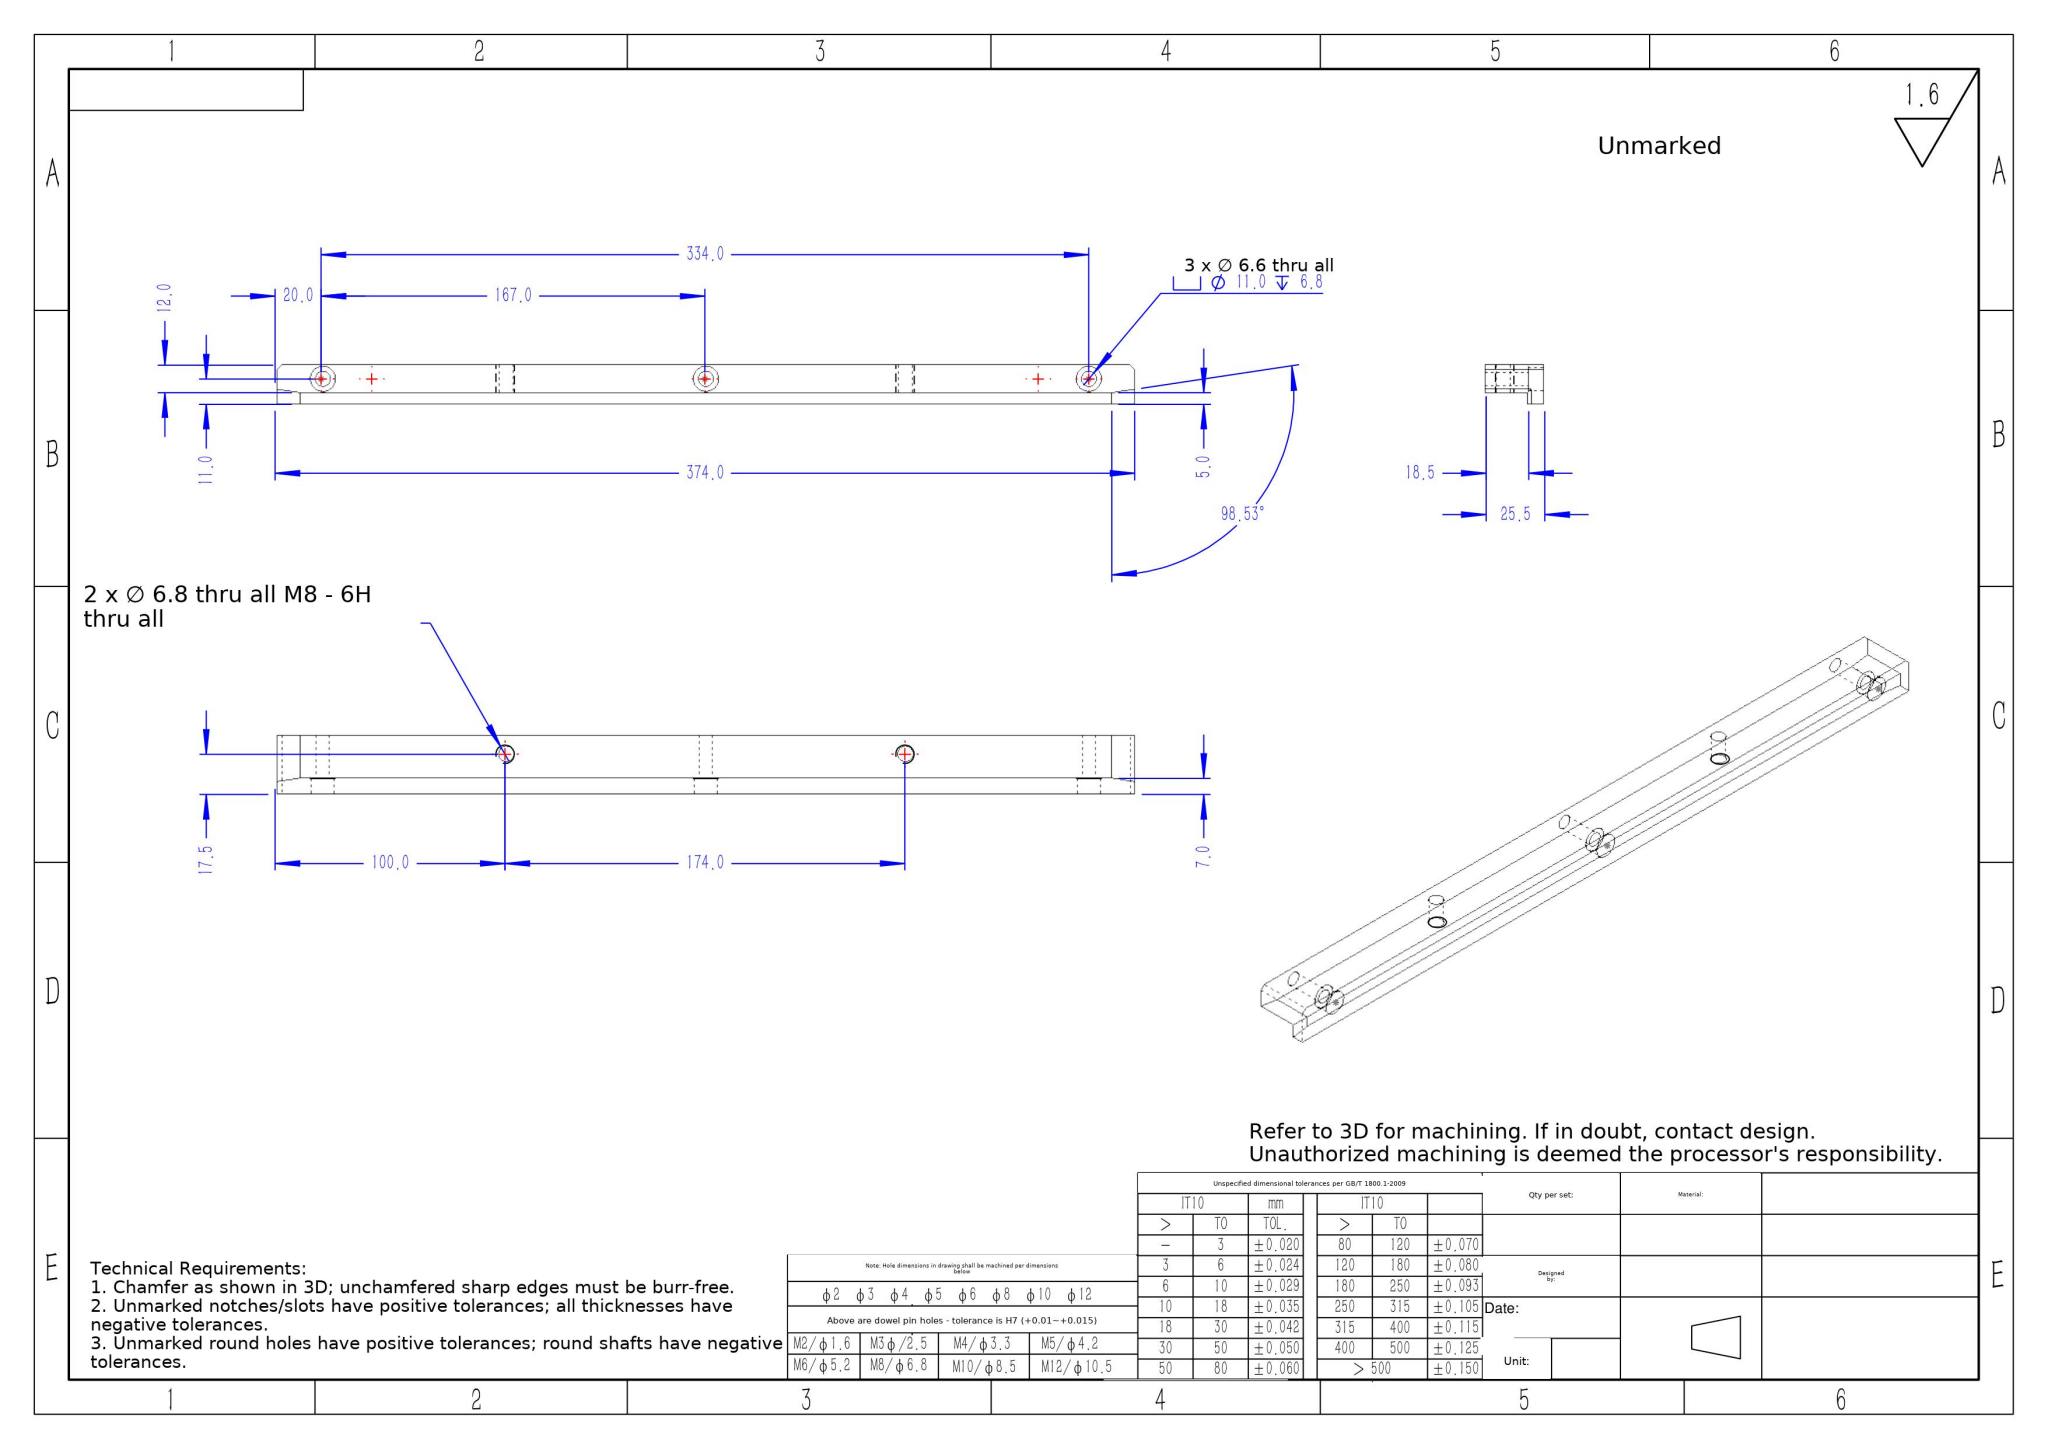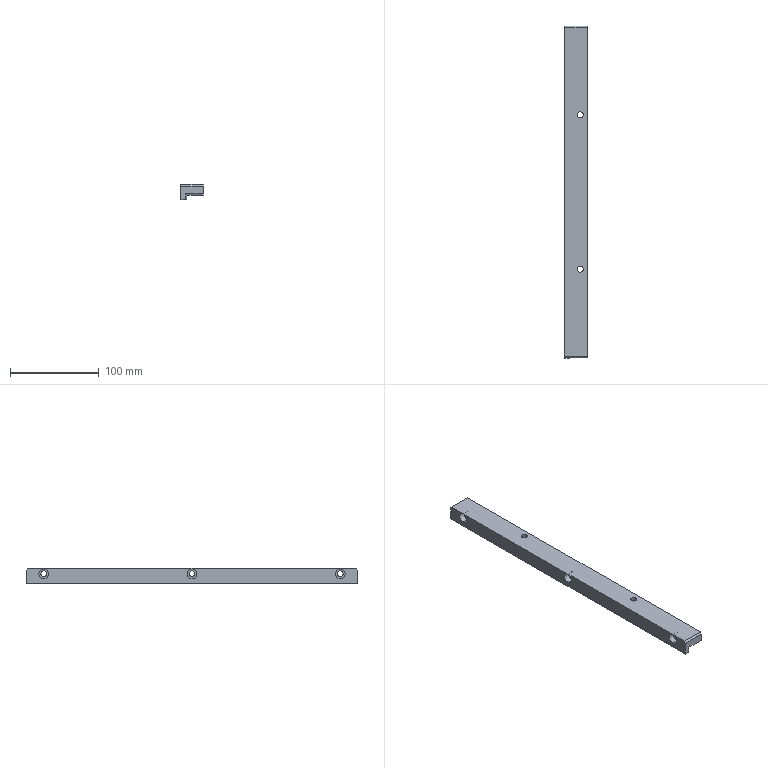Part | SolidWorks | mm | 1 solid | 33 faces | box 25.5 x 374 x 17 mm | volume 122335 mm3 | plane 17 | cylinder 16 | commonest cylinder face diameters 11 x6 6.6 x6 6.8 x4
STEP:
#1=CARTESIAN_POINT('',(14.,83.6,17.));
#2=VERTEX_POINT('',#1);
#3=CARTESIAN_POINT('',(14.,90.4,17.));
#4=VERTEX_POINT('',#3);
#5=CARTESIAN_POINT('',(14.,87.,17.));
#6=DIRECTION('',(0.,-0.,-1.));
#7=DIRECTION('',(0.,1.,0.));
#8=AXIS2_PLACEMENT_3D('',#5,#6,#7);
#9=CIRCLE('',#8,3.4);
#10=EDGE_CURVE('',#2,#4,#9,.T.);
#11=ORIENTED_EDGE('',*,*,#10,.F.);
#12=CARTESIAN_POINT('',(14.,83.6,5.));
#13=VERTEX_POINT('',#12);
#14=CARTESIAN_POINT('',(14.,83.6,5.));
#15=DIRECTION('',(0.,-0.,-1.));
#16=VECTOR('',#15,1000.);
#17=LINE('',#14,#16);
#18=EDGE_CURVE('',#2,#13,#17,.T.);
#19=ORIENTED_EDGE('',*,*,#18,.T.);
#20=CARTESIAN_POINT('',(14.,90.4,5.));
#21=VERTEX_POINT('',#20);
#22=CARTESIAN_POINT('',(14.,87.,5.));
#23=DIRECTION('',(0.,-0.,-1.));
#24=DIRECTION('',(0.,1.,0.));
#25=AXIS2_PLACEMENT_3D('',#22,#23,#24);
#26=CIRCLE('',#25,3.4);
#27=EDGE_CURVE('',#13,#21,#26,.T.);
#28=ORIENTED_EDGE('',*,*,#27,.T.);
#29=CARTESIAN_POINT('',(14.,90.4,5.));
#30=DIRECTION('',(0.,-0.,-1.));
#31=VECTOR('',#30,1000.);
#32=LINE('',#29,#31);
#33=EDGE_CURVE('',#4,#21,#32,.T.);
#34=ORIENTED_EDGE('',*,*,#33,.F.);
#35=EDGE_LOOP('',(#11,#19,#28,#34));
#36=FACE_OUTER_BOUND('',#35,.T.);
#37=CARTESIAN_POINT('',(14.,87.,5.));
#38=DIRECTION('',(0.,-0.,-1.));
#39=DIRECTION('',(0.,1.,0.));
#40=AXIS2_PLACEMENT_3D('',#37,#38,#39);
#41=CYLINDRICAL_SURFACE('',#40,3.4);
#42=ADVANCED_FACE('',(#36),#41,.F.);
#43=CARTESIAN_POINT('',(14.,-90.4,17.));
#44=VERTEX_POINT('',#43);
#45=CARTESIAN_POINT('',(14.,-83.6,17.));
#46=VERTEX_POINT('',#45);
#47=CARTESIAN_POINT('',(14.,-87.,17.));
#48=DIRECTION('',(0.,0.,-1.));
#49=DIRECTION('',(0.,1.,0.));
#50=AXIS2_PLACEMENT_3D('',#47,#48,#49);
#51=CIRCLE('',#50,3.4);
#52=EDGE_CURVE('',#44,#46,#51,.T.);
#53=ORIENTED_EDGE('',*,*,#52,.F.);
#54=CARTESIAN_POINT('',(14.,-90.4,5.));
#55=VERTEX_POINT('',#54);
#56=CARTESIAN_POINT('',(14.,-90.4,5.));
#57=DIRECTION('',(0.,0.,-1.));
#58=VECTOR('',#57,1000.);
#59=LINE('',#56,#58);
#60=EDGE_CURVE('',#44,#55,#59,.T.);
#61=ORIENTED_EDGE('',*,*,#60,.T.);
#62=CARTESIAN_POINT('',(14.,-83.6,5.));
#63=VERTEX_POINT('',#62);
#64=CARTESIAN_POINT('',(14.,-87.,5.));
#65=DIRECTION('',(0.,0.,-1.));
#66=DIRECTION('',(0.,1.,0.));
#67=AXIS2_PLACEMENT_3D('',#64,#65,#66);
#68=CIRCLE('',#67,3.4);
#69=EDGE_CURVE('',#55,#63,#68,.T.);
#70=ORIENTED_EDGE('',*,*,#69,.T.);
#71=CARTESIAN_POINT('',(14.,-83.6,5.));
#72=DIRECTION('',(0.,0.,-1.));
#73=VECTOR('',#72,1000.);
#74=LINE('',#71,#73);
#75=EDGE_CURVE('',#46,#63,#74,.T.);
#76=ORIENTED_EDGE('',*,*,#75,.F.);
#77=EDGE_LOOP('',(#53,#61,#70,#76));
#78=FACE_OUTER_BOUND('',#77,.T.);
#79=CARTESIAN_POINT('',(14.,-87.,5.));
#80=DIRECTION('',(0.,0.,-1.));
#81=DIRECTION('',(0.,1.,0.));
#82=AXIS2_PLACEMENT_3D('',#79,#80,#81);
#83=CYLINDRICAL_SURFACE('',#82,3.4);
#84=ADVANCED_FACE('',(#78),#83,.F.);
#85=CARTESIAN_POINT('',(3.3,-167.,5.5));
#86=VERTEX_POINT('',#85);
#87=CARTESIAN_POINT('',(3.3,-167.,16.5));
#88=VERTEX_POINT('',#87);
#89=CARTESIAN_POINT('',(3.3,-167.,11.));
#90=DIRECTION('',(-1.,0.,0.));
#91=DIRECTION('',(0.,0.,1.));
#92=AXIS2_PLACEMENT_3D('',#89,#90,#91);
#93=CIRCLE('',#92,5.5);
#94=EDGE_CURVE('',#86,#88,#93,.T.);
#95=ORIENTED_EDGE('',*,*,#94,.F.);
#96=CARTESIAN_POINT('',(-3.5,-167.,5.5));
#97=VERTEX_POINT('',#96);
#98=CARTESIAN_POINT('',(-3.5,-167.,5.5));
#99=DIRECTION('',(-1.,0.,0.));
#100=VECTOR('',#99,1000.);
#101=LINE('',#98,#100);
#102=EDGE_CURVE('',#86,#97,#101,.T.);
#103=ORIENTED_EDGE('',*,*,#102,.T.);
#104=CARTESIAN_POINT('',(-3.5,-167.,16.5));
#105=VERTEX_POINT('',#104);
#106=CARTESIAN_POINT('',(-3.5,-167.,11.));
#107=DIRECTION('',(-1.,0.,0.));
#108=DIRECTION('',(0.,0.,1.));
#109=AXIS2_PLACEMENT_3D('',#106,#107,#108);
#110=CIRCLE('',#109,5.5);
#111=EDGE_CURVE('',#97,#105,#110,.T.);
#112=ORIENTED_EDGE('',*,*,#111,.T.);
#113=CARTESIAN_POINT('',(-3.5,-167.,16.5));
#114=DIRECTION('',(-1.,0.,0.));
#115=VECTOR('',#114,1000.);
#116=LINE('',#113,#115);
#117=EDGE_CURVE('',#88,#105,#116,.T.);
#118=ORIENTED_EDGE('',*,*,#117,.F.);
#119=EDGE_LOOP('',(#95,#103,#112,#118));
#120=FACE_OUTER_BOUND('',#119,.T.);
#121=CARTESIAN_POINT('',(-3.5,-167.,11.));
#122=DIRECTION('',(-1.,0.,0.));
#123=DIRECTION('',(0.,0.,1.));
#124=AXIS2_PLACEMENT_3D('',#121,#122,#123);
#125=CYLINDRICAL_SURFACE('',#124,5.5);
#126=ADVANCED_FACE('',(#120),#125,.F.);
#127=CARTESIAN_POINT('',(22.,-167.,7.7));
#128=VERTEX_POINT('',#127);
#129=CARTESIAN_POINT('',(22.,-167.,14.3));
#130=VERTEX_POINT('',#129);
#131=CARTESIAN_POINT('',(22.,-167.,11.));
#132=DIRECTION('',(-1.,0.,0.));
#133=DIRECTION('',(0.,0.,1.));
#134=AXIS2_PLACEMENT_3D('',#131,#132,#133);
#135=CIRCLE('',#134,3.3);
#136=EDGE_CURVE('',#128,#130,#135,.T.);
#137=ORIENTED_EDGE('',*,*,#136,.F.);
#138=CARTESIAN_POINT('',(3.3,-167.,7.7));
#139=VERTEX_POINT('',#138);
#140=CARTESIAN_POINT('',(-3.5,-167.,7.7));
#141=DIRECTION('',(-1.,0.,0.));
#142=VECTOR('',#141,1000.);
#143=LINE('',#140,#142);
#144=EDGE_CURVE('',#128,#139,#143,.T.);
#145=ORIENTED_EDGE('',*,*,#144,.T.);
#146=CARTESIAN_POINT('',(3.3,-167.,14.3));
#147=VERTEX_POINT('',#146);
#148=CARTESIAN_POINT('',(3.3,-167.,11.));
#149=DIRECTION('',(-1.,0.,0.));
#150=DIRECTION('',(0.,0.,1.));
#151=AXIS2_PLACEMENT_3D('',#148,#149,#150);
#152=CIRCLE('',#151,3.3);
#153=EDGE_CURVE('',#139,#147,#152,.T.);
#154=ORIENTED_EDGE('',*,*,#153,.T.);
#155=CARTESIAN_POINT('',(-3.5,-167.,14.3));
#156=DIRECTION('',(-1.,0.,0.));
#157=VECTOR('',#156,1000.);
#158=LINE('',#155,#157);
#159=EDGE_CURVE('',#130,#147,#158,.T.);
#160=ORIENTED_EDGE('',*,*,#159,.F.);
#161=EDGE_LOOP('',(#137,#145,#154,#160));
#162=FACE_OUTER_BOUND('',#161,.T.);
#163=CARTESIAN_POINT('',(-3.5,-167.,11.));
#164=DIRECTION('',(-1.,0.,0.));
#165=DIRECTION('',(0.,0.,1.));
#166=AXIS2_PLACEMENT_3D('',#163,#164,#165);
#167=CYLINDRICAL_SURFACE('',#166,3.3);
#168=ADVANCED_FACE('',(#162),#167,.F.);
#169=CARTESIAN_POINT('',(3.3,0.,5.5));
#170=VERTEX_POINT('',#169);
#171=CARTESIAN_POINT('',(3.3,0.,16.5));
#172=VERTEX_POINT('',#171);
#173=CARTESIAN_POINT('',(3.3,0.,11.));
#174=DIRECTION('',(-1.,0.,0.));
#175=DIRECTION('',(0.,0.,1.));
#176=AXIS2_PLACEMENT_3D('',#173,#174,#175);
#177=CIRCLE('',#176,5.5);
#178=EDGE_CURVE('',#170,#172,#177,.T.);
#179=ORIENTED_EDGE('',*,*,#178,.F.);
#180=CARTESIAN_POINT('',(-3.5,0.,5.5));
#181=VERTEX_POINT('',#180);
#182=CARTESIAN_POINT('',(-3.5,0.,5.5));
#183=DIRECTION('',(-1.,0.,0.));
#184=VECTOR('',#183,1000.);
#185=LINE('',#182,#184);
#186=EDGE_CURVE('',#170,#181,#185,.T.);
#187=ORIENTED_EDGE('',*,*,#186,.T.);
#188=CARTESIAN_POINT('',(-3.5,0.,16.5));
#189=VERTEX_POINT('',#188);
#190=CARTESIAN_POINT('',(-3.5,0.,11.));
#191=DIRECTION('',(-1.,0.,0.));
#192=DIRECTION('',(0.,0.,1.));
#193=AXIS2_PLACEMENT_3D('',#190,#191,#192);
#194=CIRCLE('',#193,5.5);
#195=EDGE_CURVE('',#181,#189,#194,.T.);
#196=ORIENTED_EDGE('',*,*,#195,.T.);
#197=CARTESIAN_POINT('',(-3.5,0.,16.5));
#198=DIRECTION('',(-1.,0.,0.));
#199=VECTOR('',#198,1000.);
#200=LINE('',#197,#199);
#201=EDGE_CURVE('',#172,#189,#200,.T.);
#202=ORIENTED_EDGE('',*,*,#201,.F.);
#203=EDGE_LOOP('',(#179,#187,#196,#202));
#204=FACE_OUTER_BOUND('',#203,.T.);
#205=CARTESIAN_POINT('',(-3.5,0.,11.));
#206=DIRECTION('',(-1.,0.,0.));
#207=DIRECTION('',(0.,0.,1.));
#208=AXIS2_PLACEMENT_3D('',#205,#206,#207);
#209=CYLINDRICAL_SURFACE('',#208,5.5);
#210=ADVANCED_FACE('',(#204),#209,.F.);
#211=CARTESIAN_POINT('',(22.,0.,7.7));
#212=VERTEX_POINT('',#211);
#213=CARTESIAN_POINT('',(22.,0.,14.3));
#214=VERTEX_POINT('',#213);
#215=CARTESIAN_POINT('',(22.,0.,11.));
#216=DIRECTION('',(-1.,0.,0.));
#217=DIRECTION('',(0.,0.,1.));
#218=AXIS2_PLACEMENT_3D('',#215,#216,#217);
#219=CIRCLE('',#218,3.3);
#220=EDGE_CURVE('',#212,#214,#219,.T.);
#221=ORIENTED_EDGE('',*,*,#220,.F.);
#222=CARTESIAN_POINT('',(3.3,0.,7.7));
#223=VERTEX_POINT('',#222);
#224=CARTESIAN_POINT('',(-3.5,0.,7.7));
#225=DIRECTION('',(-1.,0.,0.));
#226=VECTOR('',#225,1000.);
#227=LINE('',#224,#226);
#228=EDGE_CURVE('',#212,#223,#227,.T.);
#229=ORIENTED_EDGE('',*,*,#228,.T.);
#230=CARTESIAN_POINT('',(3.3,0.,14.3));
#231=VERTEX_POINT('',#230);
#232=CARTESIAN_POINT('',(3.3,0.,11.));
#233=DIRECTION('',(-1.,0.,0.));
#234=DIRECTION('',(0.,0.,1.));
#235=AXIS2_PLACEMENT_3D('',#232,#233,#234);
#236=CIRCLE('',#235,3.3);
#237=EDGE_CURVE('',#223,#231,#236,.T.);
#238=ORIENTED_EDGE('',*,*,#237,.T.);
#239=CARTESIAN_POINT('',(-3.5,0.,14.3));
#240=DIRECTION('',(-1.,0.,0.));
#241=VECTOR('',#240,1000.);
#242=LINE('',#239,#241);
#243=EDGE_CURVE('',#214,#231,#242,.T.);
#244=ORIENTED_EDGE('',*,*,#243,.F.);
#245=EDGE_LOOP('',(#221,#229,#238,#244));
#246=FACE_OUTER_BOUND('',#245,.T.);
#247=CARTESIAN_POINT('',(-3.5,0.,11.));
#248=DIRECTION('',(-1.,0.,0.));
#249=DIRECTION('',(0.,0.,1.));
#250=AXIS2_PLACEMENT_3D('',#247,#248,#249);
#251=CYLINDRICAL_SURFACE('',#250,3.3);
#252=ADVANCED_FACE('',(#246),#251,.F.);
#253=CARTESIAN_POINT('',(3.3,167.,5.5));
#254=VERTEX_POINT('',#253);
#255=CARTESIAN_POINT('',(3.3,167.,16.5));
#256=VERTEX_POINT('',#255);
#257=CARTESIAN_POINT('',(3.3,167.,11.));
#258=DIRECTION('',(-1.,0.,0.));
#259=DIRECTION('',(0.,0.,1.));
#260=AXIS2_PLACEMENT_3D('',#257,#258,#259);
#261=CIRCLE('',#260,5.5);
#262=EDGE_CURVE('',#254,#256,#261,.T.);
#263=ORIENTED_EDGE('',*,*,#262,.F.);
#264=CARTESIAN_POINT('',(-3.5,167.,5.5));
#265=VERTEX_POINT('',#264);
#266=CARTESIAN_POINT('',(-3.5,167.,5.5));
#267=DIRECTION('',(-1.,0.,0.));
#268=VECTOR('',#267,1000.);
#269=LINE('',#266,#268);
#270=EDGE_CURVE('',#254,#265,#269,.T.);
#271=ORIENTED_EDGE('',*,*,#270,.T.);
#272=CARTESIAN_POINT('',(-3.5,167.,16.5));
#273=VERTEX_POINT('',#272);
#274=CARTESIAN_POINT('',(-3.5,167.,11.));
#275=DIRECTION('',(-1.,0.,0.));
#276=DIRECTION('',(0.,0.,1.));
#277=AXIS2_PLACEMENT_3D('',#274,#275,#276);
#278=CIRCLE('',#277,5.5);
#279=EDGE_CURVE('',#265,#273,#278,.T.);
#280=ORIENTED_EDGE('',*,*,#279,.T.);
#281=CARTESIAN_POINT('',(-3.5,167.,16.5));
#282=DIRECTION('',(-1.,0.,0.));
#283=VECTOR('',#282,1000.);
#284=LINE('',#281,#283);
#285=EDGE_CURVE('',#256,#273,#284,.T.);
#286=ORIENTED_EDGE('',*,*,#285,.F.);
#287=EDGE_LOOP('',(#263,#271,#280,#286));
#288=FACE_OUTER_BOUND('',#287,.T.);
#289=CARTESIAN_POINT('',(-3.5,167.,11.));
#290=DIRECTION('',(-1.,0.,0.));
#291=DIRECTION('',(0.,0.,1.));
#292=AXIS2_PLACEMENT_3D('',#289,#290,#291);
#293=CYLINDRICAL_SURFACE('',#292,5.5);
#294=ADVANCED_FACE('',(#288),#293,.F.);
#295=CARTESIAN_POINT('',(22.,167.,7.7));
#296=VERTEX_POINT('',#295);
#297=CARTESIAN_POINT('',(22.,167.,14.3));
#298=VERTEX_POINT('',#297);
#299=CARTESIAN_POINT('',(22.,167.,11.));
#300=DIRECTION('',(-1.,0.,0.));
#301=DIRECTION('',(0.,0.,1.));
#302=AXIS2_PLACEMENT_3D('',#299,#300,#301);
#303=CIRCLE('',#302,3.3);
#304=EDGE_CURVE('',#296,#298,#303,.T.);
#305=ORIENTED_EDGE('',*,*,#304,.F.);
#306=CARTESIAN_POINT('',(3.3,167.,7.7));
#307=VERTEX_POINT('',#306);
#308=CARTESIAN_POINT('',(-3.5,167.,7.7));
#309=DIRECTION('',(-1.,0.,0.));
#310=VECTOR('',#309,1000.);
#311=LINE('',#308,#310);
#312=EDGE_CURVE('',#296,#307,#311,.T.);
#313=ORIENTED_EDGE('',*,*,#312,.T.);
#314=CARTESIAN_POINT('',(3.3,167.,14.3));
#315=VERTEX_POINT('',#314);
#316=CARTESIAN_POINT('',(3.3,167.,11.));
#317=DIRECTION('',(-1.,0.,0.));
#318=DIRECTION('',(0.,0.,1.));
#319=AXIS2_PLACEMENT_3D('',#316,#317,#318);
#320=CIRCLE('',#319,3.3);
#321=EDGE_CURVE('',#307,#315,#320,.T.);
#322=ORIENTED_EDGE('',*,*,#321,.T.);
#323=CARTESIAN_POINT('',(-3.5,167.,14.3));
#324=DIRECTION('',(-1.,0.,0.));
#325=VECTOR('',#324,1000.);
#326=LINE('',#323,#325);
#327=EDGE_CURVE('',#298,#315,#326,.T.);
#328=ORIENTED_EDGE('',*,*,#327,.F.);
#329=EDGE_LOOP('',(#305,#313,#322,#328));
#330=FACE_OUTER_BOUND('',#329,.T.);
#331=CARTESIAN_POINT('',(-3.5,167.,11.));
#332=DIRECTION('',(-1.,0.,0.));
#333=DIRECTION('',(0.,0.,1.));
#334=AXIS2_PLACEMENT_3D('',#331,#332,#333);
#335=CYLINDRICAL_SURFACE('',#334,3.3);
#336=ADVANCED_FACE('',(#330),#335,.F.);
#337=CARTESIAN_POINT('',(3.5,-177.,0.));
#338=VERTEX_POINT('',#337);
#339=CARTESIAN_POINT('',(3.5,177.,0.));
#340=VERTEX_POINT('',#339);
#341=CARTESIAN_POINT('',(3.5,-187.,0.));
#342=DIRECTION('',(0.,1.,0.));
#343=VECTOR('',#342,1000.);
#344=LINE('',#341,#343);
#345=EDGE_CURVE('',#338,#340,#344,.T.);
#346=ORIENTED_EDGE('',*,*,#345,.T.);
#347=CARTESIAN_POINT('',(3.5,177.,5.));
#348=VERTEX_POINT('',#347);
#349=CARTESIAN_POINT('',(3.5,177.,17.));
#350=DIRECTION('',(0.,0.,1.));
#351=VECTOR('',#350,1000.);
#352=LINE('',#349,#351);
#353=EDGE_CURVE('',#340,#348,#352,.T.);
#354=ORIENTED_EDGE('',*,*,#353,.T.);
#355=CARTESIAN_POINT('',(3.5,-177.,5.));
#356=VERTEX_POINT('',#355);
#357=CARTESIAN_POINT('',(3.5,187.,5.));
#358=DIRECTION('',(0.,1.,0.));
#359=VECTOR('',#358,1000.);
#360=LINE('',#357,#359);
#361=EDGE_CURVE('',#356,#348,#360,.T.);
#362=ORIENTED_EDGE('',*,*,#361,.F.);
#363=CARTESIAN_POINT('',(3.5,-177.,17.));
#364=DIRECTION('',(0.,0.,-1.));
#365=VECTOR('',#364,1000.);
#366=LINE('',#363,#365);
#367=EDGE_CURVE('',#356,#338,#366,.T.);
#368=ORIENTED_EDGE('',*,*,#367,.T.);
#369=EDGE_LOOP('',(#346,#354,#362,#368));
#370=FACE_OUTER_BOUND('',#369,.T.);
#371=CARTESIAN_POINT('',(3.5,-187.,17.));
#372=DIRECTION('',(-1.,0.,0.));
#373=DIRECTION('',(0.,0.,1.));
#374=AXIS2_PLACEMENT_3D('',#371,#372,#373);
#375=PLANE('',#374);
#376=ADVANCED_FACE('',(#370),#375,.F.);
#377=CARTESIAN_POINT('',(-3.5,187.,15.));
#378=VERTEX_POINT('',#377);
#379=CARTESIAN_POINT('',(-3.5,187.,0.));
#380=VERTEX_POINT('',#379);
#381=CARTESIAN_POINT('',(-3.5,187.,17.));
#382=DIRECTION('',(0.,0.,-1.));
#383=VECTOR('',#382,1000.);
#384=LINE('',#381,#383);
#385=EDGE_CURVE('',#378,#380,#384,.T.);
#386=ORIENTED_EDGE('',*,*,#385,.F.);
#387=CARTESIAN_POINT('',(22.,187.,15.));
#388=VERTEX_POINT('',#387);
#389=CARTESIAN_POINT('',(-3.5,187.,15.));
#390=DIRECTION('',(1.,0.,0.));
#391=VECTOR('',#390,1000.);
#392=LINE('',#389,#391);
#393=EDGE_CURVE('',#378,#388,#392,.T.);
#394=ORIENTED_EDGE('',*,*,#393,.T.);
#395=CARTESIAN_POINT('',(22.,187.,6.5));
#396=VERTEX_POINT('',#395);
#397=CARTESIAN_POINT('',(22.,187.,17.));
#398=DIRECTION('',(0.,0.,1.));
#399=VECTOR('',#398,1000.);
#400=LINE('',#397,#399);
#401=EDGE_CURVE('',#396,#388,#400,.T.);
#402=ORIENTED_EDGE('',*,*,#401,.F.);
#403=CARTESIAN_POINT('',(2.,187.,6.5));
#404=VERTEX_POINT('',#403);
#405=CARTESIAN_POINT('',(-3.5,187.,6.5));
#406=DIRECTION('',(-1.,0.,0.));
#407=VECTOR('',#406,1000.);
#408=LINE('',#405,#407);
#409=EDGE_CURVE('',#396,#404,#408,.T.);
#410=ORIENTED_EDGE('',*,*,#409,.T.);
#411=CARTESIAN_POINT('',(2.,187.,0.));
#412=VERTEX_POINT('',#411);
#413=CARTESIAN_POINT('',(2.,187.,17.));
#414=DIRECTION('',(0.,0.,-1.));
#415=VECTOR('',#414,1000.);
#416=LINE('',#413,#415);
#417=EDGE_CURVE('',#404,#412,#416,.T.);
#418=ORIENTED_EDGE('',*,*,#417,.T.);
#419=CARTESIAN_POINT('',(-3.5,187.,0.));
#420=DIRECTION('',(-1.,0.,0.));
#421=VECTOR('',#420,1000.);
#422=LINE('',#419,#421);
#423=EDGE_CURVE('',#412,#380,#422,.T.);
#424=ORIENTED_EDGE('',*,*,#423,.T.);
#425=EDGE_LOOP('',(#386,#394,#402,#410,#418,#424));
#426=FACE_OUTER_BOUND('',#425,.T.);
#427=CARTESIAN_POINT('',(-3.5,187.,17.));
#428=DIRECTION('',(0.,-1.,0.));
#429=DIRECTION('',(0.,0.,-1.));
#430=AXIS2_PLACEMENT_3D('',#427,#428,#429);
#431=PLANE('',#430);
#432=ADVANCED_FACE('',(#426),#431,.F.);
#433=CARTESIAN_POINT('',(-3.5,-167.,11.));
#434=DIRECTION('',(-1.,0.,0.));
#435=DIRECTION('',(0.,0.,1.));
#436=AXIS2_PLACEMENT_3D('',#433,#434,#435);
#437=CIRCLE('',#436,5.5);
#438=EDGE_CURVE('',#105,#97,#437,.T.);
#439=ORIENTED_EDGE('',*,*,#438,.F.);
#440=ORIENTED_EDGE('',*,*,#111,.F.);
#441=EDGE_LOOP('',(#439,#440));
#442=FACE_BOUND('',#441,.T.);
#443=CARTESIAN_POINT('',(-3.5,0.,11.));
#444=DIRECTION('',(-1.,0.,0.));
#445=DIRECTION('',(0.,0.,1.));
#446=AXIS2_PLACEMENT_3D('',#443,#444,#445);
#447=CIRCLE('',#446,5.5);
#448=EDGE_CURVE('',#189,#181,#447,.T.);
#449=ORIENTED_EDGE('',*,*,#448,.F.);
#450=ORIENTED_EDGE('',*,*,#195,.F.);
#451=EDGE_LOOP('',(#449,#450));
#452=FACE_BOUND('',#451,.T.);
#453=CARTESIAN_POINT('',(-3.5,167.,11.));
#454=DIRECTION('',(-1.,0.,0.));
#455=DIRECTION('',(0.,0.,1.));
#456=AXIS2_PLACEMENT_3D('',#453,#454,#455);
#457=CIRCLE('',#456,5.5);
#458=EDGE_CURVE('',#273,#265,#457,.T.);
#459=ORIENTED_EDGE('',*,*,#458,.F.);
#460=ORIENTED_EDGE('',*,*,#279,.F.);
#461=EDGE_LOOP('',(#459,#460));
#462=FACE_BOUND('',#461,.T.);
#463=CARTESIAN_POINT('',(-3.5,-187.,15.));
#464=VERTEX_POINT('',#463);
#465=CARTESIAN_POINT('',(-3.5,-187.,0.));
#466=VERTEX_POINT('',#465);
#467=CARTESIAN_POINT('',(-3.5,-187.,17.));
#468=DIRECTION('',(0.,0.,-1.));
#469=VECTOR('',#468,1000.);
#470=LINE('',#467,#469);
#471=EDGE_CURVE('',#464,#466,#470,.T.);
#472=ORIENTED_EDGE('',*,*,#471,.F.);
#473=CARTESIAN_POINT('',(-3.5,-185.,17.));
#474=VERTEX_POINT('',#473);
#475=CARTESIAN_POINT('',(-3.5,-185.,17.));
#476=DIRECTION('',(0.,0.7071,0.7071));
#477=VECTOR('',#476,1000.);
#478=LINE('',#475,#477);
#479=EDGE_CURVE('',#464,#474,#478,.T.);
#480=ORIENTED_EDGE('',*,*,#479,.T.);
#481=CARTESIAN_POINT('',(-3.5,185.,17.));
#482=VERTEX_POINT('',#481);
#483=CARTESIAN_POINT('',(-3.5,-187.,17.));
#484=DIRECTION('',(0.,-1.,0.));
#485=VECTOR('',#484,1000.);
#486=LINE('',#483,#485);
#487=EDGE_CURVE('',#482,#474,#486,.T.);
#488=ORIENTED_EDGE('',*,*,#487,.F.);
#489=CARTESIAN_POINT('',(-3.5,185.,17.));
#490=DIRECTION('',(0.,0.7071,-0.7071));
#491=VECTOR('',#490,1000.);
#492=LINE('',#489,#491);
#493=EDGE_CURVE('',#482,#378,#492,.T.);
#494=ORIENTED_EDGE('',*,*,#493,.T.);
#495=ORIENTED_EDGE('',*,*,#385,.T.);
#496=CARTESIAN_POINT('',(-3.5,-187.,0.));
#497=DIRECTION('',(0.,-1.,0.));
#498=VECTOR('',#497,1000.);
#499=LINE('',#496,#498);
#500=EDGE_CURVE('',#380,#466,#499,.T.);
#501=ORIENTED_EDGE('',*,*,#500,.T.);
#502=EDGE_LOOP('',(#472,#480,#488,#494,#495,#501));
#503=FACE_OUTER_BOUND('',#502,.T.);
#504=CARTESIAN_POINT('',(-3.5,-187.,17.));
#505=DIRECTION('',(1.,0.,0.));
#506=DIRECTION('',(0.,0.,-1.));
#507=AXIS2_PLACEMENT_3D('',#504,#505,#506);
#508=PLANE('',#507);
#509=ADVANCED_FACE('',(#442,#452,#462,#503),#508,.F.);
#510=CARTESIAN_POINT('',(22.,-187.,15.));
#511=VERTEX_POINT('',#510);
#512=CARTESIAN_POINT('',(22.,-187.,6.5));
#513=VERTEX_POINT('',#512);
#514=CARTESIAN_POINT('',(22.,-187.,17.));
#515=DIRECTION('',(0.,0.,-1.));
#516=VECTOR('',#515,1000.);
#517=LINE('',#514,#516);
#518=EDGE_CURVE('',#511,#513,#517,.T.);
#519=ORIENTED_EDGE('',*,*,#518,.F.);
#520=CARTESIAN_POINT('',(-3.5,-187.,15.));
#521=DIRECTION('',(-1.,0.,0.));
#522=VECTOR('',#521,1000.);
#523=LINE('',#520,#522);
#524=EDGE_CURVE('',#511,#464,#523,.T.);
#525=ORIENTED_EDGE('',*,*,#524,.T.);
#526=ORIENTED_EDGE('',*,*,#471,.T.);
#527=CARTESIAN_POINT('',(2.,-187.,0.));
#528=VERTEX_POINT('',#527);
#529=CARTESIAN_POINT('',(-3.5,-187.,0.));
#530=DIRECTION('',(1.,0.,0.));
#531=VECTOR('',#530,1000.);
#532=LINE('',#529,#531);
#533=EDGE_CURVE('',#466,#528,#532,.T.);
#534=ORIENTED_EDGE('',*,*,#533,.T.);
#535=CARTESIAN_POINT('',(2.,-187.,6.5));
#536=VERTEX_POINT('',#535);
#537=CARTESIAN_POINT('',(2.,-187.,17.));
#538=DIRECTION('',(0.,0.,1.));
#539=VECTOR('',#538,1000.);
#540=LINE('',#537,#539);
#541=EDGE_CURVE('',#528,#536,#540,.T.);
#542=ORIENTED_EDGE('',*,*,#541,.T.);
#543=CARTESIAN_POINT('',(-3.5,-187.,6.5));
#544=DIRECTION('',(1.,0.,0.));
#545=VECTOR('',#544,1000.);
#546=LINE('',#543,#545);
#547=EDGE_CURVE('',#536,#513,#546,.T.);
#548=ORIENTED_EDGE('',*,*,#547,.T.);
#549=EDGE_LOOP('',(#519,#525,#526,#534,#542,#548));
#550=FACE_OUTER_BOUND('',#549,.T.);
#551=CARTESIAN_POINT('',(-3.5,-187.,17.));
#552=DIRECTION('',(0.,1.,0.));
#553=DIRECTION('',(0.,0.,1.));
#554=AXIS2_PLACEMENT_3D('',#551,#552,#553);
#555=PLANE('',#554);
#556=ADVANCED_FACE('',(#550),#555,.F.);
#557=CARTESIAN_POINT('',(14.,87.,17.));
#558=DIRECTION('',(0.,-0.,-1.));
#559=DIRECTION('',(0.,1.,0.));
#560=AXIS2_PLACEMENT_3D('',#557,#558,#559);
#561=CIRCLE('',#560,3.4);
#562=EDGE_CURVE('',#4,#2,#561,.T.);
#563=ORIENTED_EDGE('',*,*,#562,.T.);
#564=ORIENTED_EDGE('',*,*,#10,.T.);
#565=EDGE_LOOP('',(#563,#564));
#566=FACE_BOUND('',#565,.T.);
#567=CARTESIAN_POINT('',(14.,-87.,17.));
#568=DIRECTION('',(0.,0.,-1.));
#569=DIRECTION('',(0.,1.,0.));
#570=AXIS2_PLACEMENT_3D('',#567,#568,#569);
#571=CIRCLE('',#570,3.4);
#572=EDGE_CURVE('',#46,#44,#571,.T.);
#573=ORIENTED_EDGE('',*,*,#572,.T.);
#574=ORIENTED_EDGE('',*,*,#52,.T.);
#575=EDGE_LOOP('',(#573,#574));
#576=FACE_BOUND('',#575,.T.);
#577=ORIENTED_EDGE('',*,*,#487,.T.);
#578=CARTESIAN_POINT('',(22.,-185.,17.));
#579=VERTEX_POINT('',#578);
#580=CARTESIAN_POINT('',(0.,-185.,17.));
#581=DIRECTION('',(1.,0.,0.));
#582=VECTOR('',#581,1000.);
#583=LINE('',#580,#582);
#584=EDGE_CURVE('',#474,#579,#583,.T.);
#585=ORIENTED_EDGE('',*,*,#584,.T.);
#586=CARTESIAN_POINT('',(22.,185.,17.));
#587=VERTEX_POINT('',#586);
#588=CARTESIAN_POINT('',(22.,187.,17.));
#589=DIRECTION('',(0.,-1.,-0.));
#590=VECTOR('',#589,1000.);
#591=LINE('',#588,#590);
#592=EDGE_CURVE('',#587,#579,#591,.T.);
#593=ORIENTED_EDGE('',*,*,#592,.F.);
#594=CARTESIAN_POINT('',(0.,185.,17.));
#595=DIRECTION('',(-1.,0.,0.));
#596=VECTOR('',#595,1000.);
#597=LINE('',#594,#596);
#598=EDGE_CURVE('',#587,#482,#597,.T.);
#599=ORIENTED_EDGE('',*,*,#598,.T.);
#600=EDGE_LOOP('',(#577,#585,#593,#599));
#601=FACE_OUTER_BOUND('',#600,.T.);
#602=CARTESIAN_POINT('',(0.,0.,17.));
#603=DIRECTION('',(0.,0.,-1.));
#604=DIRECTION('',(-1.,0.,0.));
#605=AXIS2_PLACEMENT_3D('',#602,#603,#604);
#606=PLANE('',#605);
#607=ADVANCED_FACE('',(#566,#576,#601),#606,.F.);
#608=ORIENTED_EDGE('',*,*,#423,.F.);
#609=CARTESIAN_POINT('',(29.389,4.408,0.));
#610=DIRECTION('',(0.1483,-0.9889,0.));
#611=VECTOR('',#610,1000.);
#612=LINE('',#609,#611);
#613=EDGE_CURVE('',#412,#340,#612,.T.);
#614=ORIENTED_EDGE('',*,*,#613,.T.);
#615=ORIENTED_EDGE('',*,*,#345,.F.);
#616=CARTESIAN_POINT('',(29.389,-4.408,0.));
#617=DIRECTION('',(-0.1483,-0.9889,0.));
#618=VECTOR('',#617,1000.);
#619=LINE('',#616,#618);
#620=EDGE_CURVE('',#338,#528,#619,.T.);
#621=ORIENTED_EDGE('',*,*,#620,.T.);
#622=ORIENTED_EDGE('',*,*,#533,.F.);
#623=ORIENTED_EDGE('',*,*,#500,.F.);
#624=EDGE_LOOP('',(#608,#614,#615,#621,#622,#623));
#625=FACE_OUTER_BOUND('',#624,.T.);
#626=CARTESIAN_POINT('',(0.,0.,0.));
#627=DIRECTION('',(0.,0.,-1.));
#628=DIRECTION('',(-1.,0.,0.));
#629=AXIS2_PLACEMENT_3D('',#626,#627,#628);
#630=PLANE('',#629);
#631=ADVANCED_FACE('',(#625),#630,.T.);
#632=CARTESIAN_POINT('',(14.,87.,5.));
#633=DIRECTION('',(0.,-0.,-1.));
#634=DIRECTION('',(0.,1.,0.));
#635=AXIS2_PLACEMENT_3D('',#632,#633,#634);
#636=CIRCLE('',#635,3.4);
#637=EDGE_CURVE('',#21,#13,#636,.T.);
#638=ORIENTED_EDGE('',*,*,#637,.F.);
#639=ORIENTED_EDGE('',*,*,#27,.F.);
#640=EDGE_LOOP('',(#638,#639));
#641=FACE_BOUND('',#640,.T.);
#642=CARTESIAN_POINT('',(14.,-87.,5.));
#643=DIRECTION('',(0.,0.,-1.));
#644=DIRECTION('',(0.,1.,0.));
#645=AXIS2_PLACEMENT_3D('',#642,#643,#644);
#646=CIRCLE('',#645,3.4);
#647=EDGE_CURVE('',#63,#55,#646,.T.);
#648=ORIENTED_EDGE('',*,*,#647,.F.);
#649=ORIENTED_EDGE('',*,*,#69,.F.);
#650=EDGE_LOOP('',(#648,#649));
#651=FACE_BOUND('',#650,.T.);
#652=ORIENTED_EDGE('',*,*,#361,.T.);
#653=CARTESIAN_POINT('',(22.,177.,5.));
#654=VERTEX_POINT('',#653);
#655=CARTESIAN_POINT('',(22.,177.,5.));
#656=DIRECTION('',(1.,0.,0.));
#657=VECTOR('',#656,1000.);
#658=LINE('',#655,#657);
#659=EDGE_CURVE('',#348,#654,#658,.T.);
#660=ORIENTED_EDGE('',*,*,#659,.T.);
#661=CARTESIAN_POINT('',(22.,-177.,5.));
#662=VERTEX_POINT('',#661);
#663=CARTESIAN_POINT('',(22.,187.,5.));
#664=DIRECTION('',(0.,1.,0.));
#665=VECTOR('',#664,1000.);
#666=LINE('',#663,#665);
#667=EDGE_CURVE('',#662,#654,#666,.T.);
#668=ORIENTED_EDGE('',*,*,#667,.F.);
#669=CARTESIAN_POINT('',(22.,-177.,5.));
#670=DIRECTION('',(-1.,0.,0.));
#671=VECTOR('',#670,1000.);
#672=LINE('',#669,#671);
#673=EDGE_CURVE('',#662,#356,#672,.T.);
#674=ORIENTED_EDGE('',*,*,#673,.T.);
#675=EDGE_LOOP('',(#652,#660,#668,#674));
#676=FACE_OUTER_BOUND('',#675,.T.);
#677=CARTESIAN_POINT('',(22.,187.,5.));
#678=DIRECTION('',(0.,-0.,1.));
#679=DIRECTION('',(0.,-1.,-0.));
#680=AXIS2_PLACEMENT_3D('',#677,#678,#679);
#681=PLANE('',#680);
#682=ADVANCED_FACE('',(#641,#651,#676),#681,.F.);
#683=CARTESIAN_POINT('',(22.,-167.,11.));
#684=DIRECTION('',(-1.,0.,0.));
#685=DIRECTION('',(0.,0.,1.));
#686=AXIS2_PLACEMENT_3D('',#683,#684,#685);
#687=CIRCLE('',#686,3.3);
#688=EDGE_CURVE('',#130,#128,#687,.T.);
#689=ORIENTED_EDGE('',*,*,#688,.T.);
#690=ORIENTED_EDGE('',*,*,#136,.T.);
#691=EDGE_LOOP('',(#689,#690));
#692=FACE_BOUND('',#691,.T.);
#693=CARTESIAN_POINT('',(22.,0.,11.));
#694=DIRECTION('',(-1.,0.,0.));
#695=DIRECTION('',(0.,0.,1.));
#696=AXIS2_PLACEMENT_3D('',#693,#694,#695);
#697=CIRCLE('',#696,3.3);
#698=EDGE_CURVE('',#214,#212,#697,.T.);
#699=ORIENTED_EDGE('',*,*,#698,.T.);
#700=ORIENTED_EDGE('',*,*,#220,.T.);
#701=EDGE_LOOP('',(#699,#700));
#702=FACE_BOUND('',#701,.T.);
#703=CARTESIAN_POINT('',(22.,167.,11.));
#704=DIRECTION('',(-1.,0.,0.));
#705=DIRECTION('',(0.,0.,1.));
#706=AXIS2_PLACEMENT_3D('',#703,#704,#705);
#707=CIRCLE('',#706,3.3);
#708=EDGE_CURVE('',#298,#296,#707,.T.);
#709=ORIENTED_EDGE('',*,*,#708,.T.);
#710=ORIENTED_EDGE('',*,*,#304,.T.);
#711=EDGE_LOOP('',(#709,#710));
#712=FACE_BOUND('',#711,.T.);
#713=ORIENTED_EDGE('',*,*,#592,.T.);
#714=CARTESIAN_POINT('',(22.,-101.,101.));
#715=DIRECTION('',(0.,-0.7071,-0.7071));
#716=VECTOR('',#715,1000.);
#717=LINE('',#714,#716);
#718=EDGE_CURVE('',#579,#511,#717,.T.);
#719=ORIENTED_EDGE('',*,*,#718,.T.);
#720=ORIENTED_EDGE('',*,*,#518,.T.);
#721=CARTESIAN_POINT('',(22.,-3.161,-21.076));
#722=DIRECTION('',(0.,0.9889,-0.1483));
#723=VECTOR('',#722,1000.);
#724=LINE('',#721,#723);
#725=EDGE_CURVE('',#513,#662,#724,.T.);
#726=ORIENTED_EDGE('',*,*,#725,.T.);
#727=ORIENTED_EDGE('',*,*,#667,.T.);
#728=CARTESIAN_POINT('',(22.,3.161,-21.076));
#729=DIRECTION('',(0.,0.9889,0.1483));
#730=VECTOR('',#729,1000.);
#731=LINE('',#728,#730);
#732=EDGE_CURVE('',#654,#396,#731,.T.);
#733=ORIENTED_EDGE('',*,*,#732,.T.);
#734=ORIENTED_EDGE('',*,*,#401,.T.);
#735=CARTESIAN_POINT('',(22.,101.,101.));
#736=DIRECTION('',(0.,-0.7071,0.7071));
#737=VECTOR('',#736,1000.);
#738=LINE('',#735,#737);
#739=EDGE_CURVE('',#388,#587,#738,.T.);
#740=ORIENTED_EDGE('',*,*,#739,.T.);
#741=EDGE_LOOP('',(#713,#719,#720,#726,#727,#733,#734,#740));
#742=FACE_OUTER_BOUND('',#741,.T.);
#743=CARTESIAN_POINT('',(22.,0.,0.));
#744=DIRECTION('',(1.,0.,0.));
#745=DIRECTION('',(0.,0.,-1.));
#746=AXIS2_PLACEMENT_3D('',#743,#744,#745);
#747=PLANE('',#746);
#748=ADVANCED_FACE('',(#692,#702,#712,#742),#747,.T.);
#749=ORIENTED_EDGE('',*,*,#312,.F.);
#750=ORIENTED_EDGE('',*,*,#708,.F.);
#751=ORIENTED_EDGE('',*,*,#327,.T.);
#752=CARTESIAN_POINT('',(3.3,167.,11.));
#753=DIRECTION('',(-1.,0.,0.));
#754=DIRECTION('',(0.,0.,1.));
#755=AXIS2_PLACEMENT_3D('',#752,#753,#754);
#756=CIRCLE('',#755,3.3);
#757=EDGE_CURVE('',#315,#307,#756,.T.);
#758=ORIENTED_EDGE('',*,*,#757,.T.);
#759=EDGE_LOOP('',(#749,#750,#751,#758));
#760=FACE_OUTER_BOUND('',#759,.T.);
#761=CARTESIAN_POINT('',(-3.5,167.,11.));
#762=DIRECTION('',(-1.,0.,0.));
#763=DIRECTION('',(0.,0.,1.));
#764=AXIS2_PLACEMENT_3D('',#761,#762,#763);
#765=CYLINDRICAL_SURFACE('',#764,3.3);
#766=ADVANCED_FACE('',(#760),#765,.F.);
#767=ORIENTED_EDGE('',*,*,#757,.F.);
#768=ORIENTED_EDGE('',*,*,#321,.F.);
#769=EDGE_LOOP('',(#767,#768));
#770=FACE_BOUND('',#769,.T.);
#771=CARTESIAN_POINT('',(3.3,167.,11.));
#772=DIRECTION('',(-1.,0.,0.));
#773=DIRECTION('',(0.,0.,1.));
#774=AXIS2_PLACEMENT_3D('',#771,#772,#773);
#775=CIRCLE('',#774,5.5);
#776=EDGE_CURVE('',#256,#254,#775,.T.);
#777=ORIENTED_EDGE('',*,*,#776,.T.);
#778=ORIENTED_EDGE('',*,*,#262,.T.);
#779=EDGE_LOOP('',(#777,#778));
#780=FACE_OUTER_BOUND('',#779,.T.);
#781=CARTESIAN_POINT('',(3.3,170.3,11.));
#782=DIRECTION('',(1.,0.,0.));
#783=DIRECTION('',(0.,0.,-1.));
#784=AXIS2_PLACEMENT_3D('',#781,#782,#783);
#785=PLANE('',#784);
#786=ADVANCED_FACE('',(#770,#780),#785,.F.);
#787=ORIENTED_EDGE('',*,*,#270,.F.);
#788=ORIENTED_EDGE('',*,*,#776,.F.);
#789=ORIENTED_EDGE('',*,*,#285,.T.);
#790=ORIENTED_EDGE('',*,*,#458,.T.);
#791=EDGE_LOOP('',(#787,#788,#789,#790));
#792=FACE_OUTER_BOUND('',#791,.T.);
#793=CARTESIAN_POINT('',(-3.5,167.,11.));
#794=DIRECTION('',(-1.,0.,0.));
#795=DIRECTION('',(0.,0.,1.));
#796=AXIS2_PLACEMENT_3D('',#793,#794,#795);
#797=CYLINDRICAL_SURFACE('',#796,5.5);
#798=ADVANCED_FACE('',(#792),#797,.F.);
#799=ORIENTED_EDGE('',*,*,#228,.F.);
#800=ORIENTED_EDGE('',*,*,#698,.F.);
#801=ORIENTED_EDGE('',*,*,#243,.T.);
#802=CARTESIAN_POINT('',(3.3,0.,11.));
#803=DIRECTION('',(-1.,0.,0.));
#804=DIRECTION('',(0.,0.,1.));
#805=AXIS2_PLACEMENT_3D('',#802,#803,#804);
#806=CIRCLE('',#805,3.3);
#807=EDGE_CURVE('',#231,#223,#806,.T.);
#808=ORIENTED_EDGE('',*,*,#807,.T.);
#809=EDGE_LOOP('',(#799,#800,#801,#808));
#810=FACE_OUTER_BOUND('',#809,.T.);
#811=CARTESIAN_POINT('',(-3.5,0.,11.));
#812=DIRECTION('',(-1.,0.,0.));
#813=DIRECTION('',(0.,0.,1.));
#814=AXIS2_PLACEMENT_3D('',#811,#812,#813);
#815=CYLINDRICAL_SURFACE('',#814,3.3);
#816=ADVANCED_FACE('',(#810),#815,.F.);
#817=ORIENTED_EDGE('',*,*,#807,.F.);
#818=ORIENTED_EDGE('',*,*,#237,.F.);
#819=EDGE_LOOP('',(#817,#818));
#820=FACE_BOUND('',#819,.T.);
#821=CARTESIAN_POINT('',(3.3,0.,11.));
#822=DIRECTION('',(-1.,0.,0.));
#823=DIRECTION('',(0.,0.,1.));
#824=AXIS2_PLACEMENT_3D('',#821,#822,#823);
#825=CIRCLE('',#824,5.5);
#826=EDGE_CURVE('',#172,#170,#825,.T.);
#827=ORIENTED_EDGE('',*,*,#826,.T.);
#828=ORIENTED_EDGE('',*,*,#178,.T.);
#829=EDGE_LOOP('',(#827,#828));
#830=FACE_OUTER_BOUND('',#829,.T.);
#831=CARTESIAN_POINT('',(3.3,3.3,11.));
#832=DIRECTION('',(1.,0.,0.));
#833=DIRECTION('',(0.,0.,-1.));
#834=AXIS2_PLACEMENT_3D('',#831,#832,#833);
#835=PLANE('',#834);
#836=ADVANCED_FACE('',(#820,#830),#835,.F.);
#837=ORIENTED_EDGE('',*,*,#186,.F.);
#838=ORIENTED_EDGE('',*,*,#826,.F.);
#839=ORIENTED_EDGE('',*,*,#201,.T.);
#840=ORIENTED_EDGE('',*,*,#448,.T.);
#841=EDGE_LOOP('',(#837,#838,#839,#840));
#842=FACE_OUTER_BOUND('',#841,.T.);
#843=CARTESIAN_POINT('',(-3.5,0.,11.));
#844=DIRECTION('',(-1.,0.,0.));
#845=DIRECTION('',(0.,0.,1.));
#846=AXIS2_PLACEMENT_3D('',#843,#844,#845);
#847=CYLINDRICAL_SURFACE('',#846,5.5);
#848=ADVANCED_FACE('',(#842),#847,.F.);
#849=ORIENTED_EDGE('',*,*,#144,.F.);
#850=ORIENTED_EDGE('',*,*,#688,.F.);
#851=ORIENTED_EDGE('',*,*,#159,.T.);
#852=CARTESIAN_POINT('',(3.3,-167.,11.));
#853=DIRECTION('',(-1.,0.,0.));
#854=DIRECTION('',(0.,0.,1.));
#855=AXIS2_PLACEMENT_3D('',#852,#853,#854);
#856=CIRCLE('',#855,3.3);
#857=EDGE_CURVE('',#147,#139,#856,.T.);
#858=ORIENTED_EDGE('',*,*,#857,.T.);
#859=EDGE_LOOP('',(#849,#850,#851,#858));
#860=FACE_OUTER_BOUND('',#859,.T.);
#861=CARTESIAN_POINT('',(-3.5,-167.,11.));
#862=DIRECTION('',(-1.,0.,0.));
#863=DIRECTION('',(0.,0.,1.));
#864=AXIS2_PLACEMENT_3D('',#861,#862,#863);
#865=CYLINDRICAL_SURFACE('',#864,3.3);
#866=ADVANCED_FACE('',(#860),#865,.F.);
#867=ORIENTED_EDGE('',*,*,#857,.F.);
#868=ORIENTED_EDGE('',*,*,#153,.F.);
#869=EDGE_LOOP('',(#867,#868));
#870=FACE_BOUND('',#869,.T.);
#871=CARTESIAN_POINT('',(3.3,-167.,11.));
#872=DIRECTION('',(-1.,0.,0.));
#873=DIRECTION('',(0.,0.,1.));
#874=AXIS2_PLACEMENT_3D('',#871,#872,#873);
#875=CIRCLE('',#874,5.5);
#876=EDGE_CURVE('',#88,#86,#875,.T.);
#877=ORIENTED_EDGE('',*,*,#876,.T.);
#878=ORIENTED_EDGE('',*,*,#94,.T.);
#879=EDGE_LOOP('',(#877,#878));
#880=FACE_OUTER_BOUND('',#879,.T.);
#881=CARTESIAN_POINT('',(3.3,-163.7,11.));
#882=DIRECTION('',(1.,0.,0.));
#883=DIRECTION('',(0.,0.,-1.));
#884=AXIS2_PLACEMENT_3D('',#881,#882,#883);
#885=PLANE('',#884);
#886=ADVANCED_FACE('',(#870,#880),#885,.F.);
#887=ORIENTED_EDGE('',*,*,#102,.F.);
#888=ORIENTED_EDGE('',*,*,#876,.F.);
#889=ORIENTED_EDGE('',*,*,#117,.T.);
#890=ORIENTED_EDGE('',*,*,#438,.T.);
#891=EDGE_LOOP('',(#887,#888,#889,#890));
#892=FACE_OUTER_BOUND('',#891,.T.);
#893=CARTESIAN_POINT('',(-3.5,-167.,11.));
#894=DIRECTION('',(-1.,0.,0.));
#895=DIRECTION('',(0.,0.,1.));
#896=AXIS2_PLACEMENT_3D('',#893,#894,#895);
#897=CYLINDRICAL_SURFACE('',#896,5.5);
#898=ADVANCED_FACE('',(#892),#897,.F.);
#899=ORIENTED_EDGE('',*,*,#725,.F.);
#900=ORIENTED_EDGE('',*,*,#547,.F.);
#901=CARTESIAN_POINT('',(3.242,-178.722,5.258));
#902=DIRECTION('',(-0.1467,-0.9782,0.1467));
#903=VECTOR('',#902,1000.);
#904=LINE('',#901,#903);
#905=EDGE_CURVE('',#356,#536,#904,.T.);
#906=ORIENTED_EDGE('',*,*,#905,.F.);
#907=ORIENTED_EDGE('',*,*,#673,.F.);
#908=EDGE_LOOP('',(#899,#900,#906,#907));
#909=FACE_OUTER_BOUND('',#908,.T.);
#910=CARTESIAN_POINT('',(22.,-177.,5.));
#911=DIRECTION('',(0.,0.1483,0.9889));
#912=DIRECTION('',(-1.,0.,0.));
#913=AXIS2_PLACEMENT_3D('',#910,#911,#912);
#914=PLANE('',#913);
#915=ADVANCED_FACE('',(#909),#914,.F.);
#916=ORIENTED_EDGE('',*,*,#905,.T.);
#917=ORIENTED_EDGE('',*,*,#541,.F.);
#918=ORIENTED_EDGE('',*,*,#620,.F.);
#919=ORIENTED_EDGE('',*,*,#367,.F.);
#920=EDGE_LOOP('',(#916,#917,#918,#919));
#921=FACE_OUTER_BOUND('',#920,.T.);
#922=CARTESIAN_POINT('',(3.5,-177.,17.));
#923=DIRECTION('',(-0.9889,0.1483,0.));
#924=DIRECTION('',(0.,0.,-1.));
#925=AXIS2_PLACEMENT_3D('',#922,#923,#924);
#926=PLANE('',#925);
#927=ADVANCED_FACE('',(#921),#926,.F.);
#928=ORIENTED_EDGE('',*,*,#732,.F.);
#929=ORIENTED_EDGE('',*,*,#659,.F.);
#930=CARTESIAN_POINT('',(1.774,188.507,6.726));
#931=DIRECTION('',(0.1467,-0.9782,-0.1467));
#932=VECTOR('',#931,1000.);
#933=LINE('',#930,#932);
#934=EDGE_CURVE('',#404,#348,#933,.T.);
#935=ORIENTED_EDGE('',*,*,#934,.F.);
#936=ORIENTED_EDGE('',*,*,#409,.F.);
#937=EDGE_LOOP('',(#928,#929,#935,#936));
#938=FACE_OUTER_BOUND('',#937,.T.);
#939=CARTESIAN_POINT('',(-3.5,187.,6.5));
#940=DIRECTION('',(0.,-0.1483,0.9889));
#941=DIRECTION('',(-1.,0.,0.));
#942=AXIS2_PLACEMENT_3D('',#939,#940,#941);
#943=PLANE('',#942);
#944=ADVANCED_FACE('',(#938),#943,.F.);
#945=ORIENTED_EDGE('',*,*,#934,.T.);
#946=ORIENTED_EDGE('',*,*,#353,.F.);
#947=ORIENTED_EDGE('',*,*,#613,.F.);
#948=ORIENTED_EDGE('',*,*,#417,.F.);
#949=EDGE_LOOP('',(#945,#946,#947,#948));
#950=FACE_OUTER_BOUND('',#949,.T.);
#951=CARTESIAN_POINT('',(2.,187.,17.));
#952=DIRECTION('',(-0.9889,-0.1483,0.));
#953=DIRECTION('',(0.,0.,-1.));
#954=AXIS2_PLACEMENT_3D('',#951,#952,#953);
#955=PLANE('',#954);
#956=ADVANCED_FACE('',(#950),#955,.F.);
#957=ORIENTED_EDGE('',*,*,#60,.F.);
#958=ORIENTED_EDGE('',*,*,#572,.F.);
#959=ORIENTED_EDGE('',*,*,#75,.T.);
#960=ORIENTED_EDGE('',*,*,#647,.T.);
#961=EDGE_LOOP('',(#957,#958,#959,#960));
#962=FACE_OUTER_BOUND('',#961,.T.);
#963=CARTESIAN_POINT('',(14.,-87.,5.));
#964=DIRECTION('',(0.,0.,-1.));
#965=DIRECTION('',(0.,1.,0.));
#966=AXIS2_PLACEMENT_3D('',#963,#964,#965);
#967=CYLINDRICAL_SURFACE('',#966,3.4);
#968=ADVANCED_FACE('',(#962),#967,.F.);
#969=ORIENTED_EDGE('',*,*,#18,.F.);
#970=ORIENTED_EDGE('',*,*,#562,.F.);
#971=ORIENTED_EDGE('',*,*,#33,.T.);
#972=ORIENTED_EDGE('',*,*,#637,.T.);
#973=EDGE_LOOP('',(#969,#970,#971,#972));
#974=FACE_OUTER_BOUND('',#973,.T.);
#975=CARTESIAN_POINT('',(14.,87.,5.));
#976=DIRECTION('',(0.,-0.,-1.));
#977=DIRECTION('',(0.,1.,0.));
#978=AXIS2_PLACEMENT_3D('',#975,#976,#977);
#979=CYLINDRICAL_SURFACE('',#978,3.4);
#980=ADVANCED_FACE('',(#974),#979,.F.);
#981=ORIENTED_EDGE('',*,*,#479,.F.);
#982=ORIENTED_EDGE('',*,*,#524,.F.);
#983=ORIENTED_EDGE('',*,*,#718,.F.);
#984=ORIENTED_EDGE('',*,*,#584,.F.);
#985=EDGE_LOOP('',(#981,#982,#983,#984));
#986=FACE_OUTER_BOUND('',#985,.T.);
#987=CARTESIAN_POINT('',(0.,-185.,17.));
#988=DIRECTION('',(0.,0.7071,-0.7071));
#989=DIRECTION('',(1.,0.,0.));
#990=AXIS2_PLACEMENT_3D('',#987,#988,#989);
#991=PLANE('',#990);
#992=ADVANCED_FACE('',(#986),#991,.F.);
#993=ORIENTED_EDGE('',*,*,#739,.F.);
#994=ORIENTED_EDGE('',*,*,#393,.F.);
#995=ORIENTED_EDGE('',*,*,#493,.F.);
#996=ORIENTED_EDGE('',*,*,#598,.F.);
#997=EDGE_LOOP('',(#993,#994,#995,#996));
#998=FACE_OUTER_BOUND('',#997,.T.);
#999=CARTESIAN_POINT('',(0.,185.,17.));
#1000=DIRECTION('',(0.,-0.7071,-0.7071));
#1001=DIRECTION('',(-1.,0.,0.));
#1002=AXIS2_PLACEMENT_3D('',#999,#1000,#1001);
#1003=PLANE('',#1002);
#1004=ADVANCED_FACE('',(#998),#1003,.F.);
#1005=CLOSED_SHELL('',(#42,#84,#126,#168,#210,#252,#294,#336,#376,#432,#509,#556,#607,#631,#682,#748,#766,#786,#798,#816,#836,#848,#866,#886,#898,#915,#927,#944,#956,#968,#980,#992,#1004));
#1006=MANIFOLD_SOLID_BREP('',#1005);
#1007=CARTESIAN_POINT('',(0.,0.,0.));
#1008=DIRECTION('',(0.,0.,1.));
#1009=DIRECTION('',(1.,0.,0.));
#1010=AXIS2_PLACEMENT_3D('',#1007,#1008,#1009);
#1011=(LENGTH_UNIT()NAMED_UNIT(*)SI_UNIT(.MILLI.,.METRE.));
#1012=UNCERTAINTY_MEASURE_WITH_UNIT(LENGTH_MEASURE(0.00001),#1011,'','');
#1013=(NAMED_UNIT(*)PLANE_ANGLE_UNIT()SI_UNIT($,.RADIAN.));
#1014=(NAMED_UNIT(*)SI_UNIT($,.STERADIAN.)SOLID_ANGLE_UNIT());
#1015=(GEOMETRIC_REPRESENTATION_CONTEXT(3)GLOBAL_UNCERTAINTY_ASSIGNED_CONTEXT((#1012))GLOBAL_UNIT_ASSIGNED_CONTEXT((#1011,#1013,#1014))REPRESENTATION_CONTEXT('',''));
#1016=ADVANCED_BREP_SHAPE_REPRESENTATION('',(#1006,#1010),#1015);